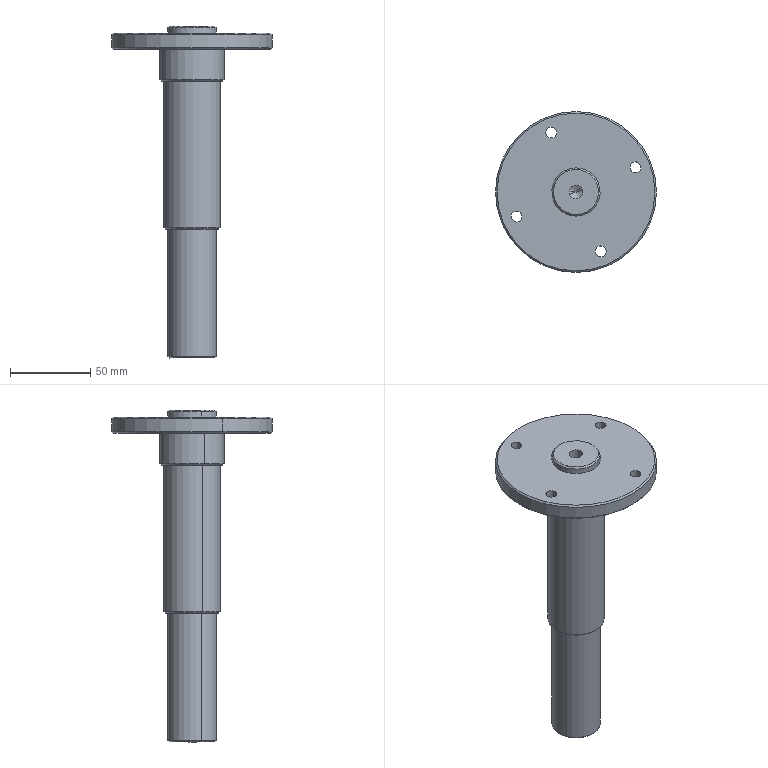Component | SolidWorks | CuttingAxis-1 | 1 solid | 44 faces | volume 246900 mm3 | cylinder 22 | cone 16 | plane 6 | commonest cylinder face diameters 6.8 x8 8.5 x4 30 x4 35 x2 40 x2 100 x2 | material Stainless Steel